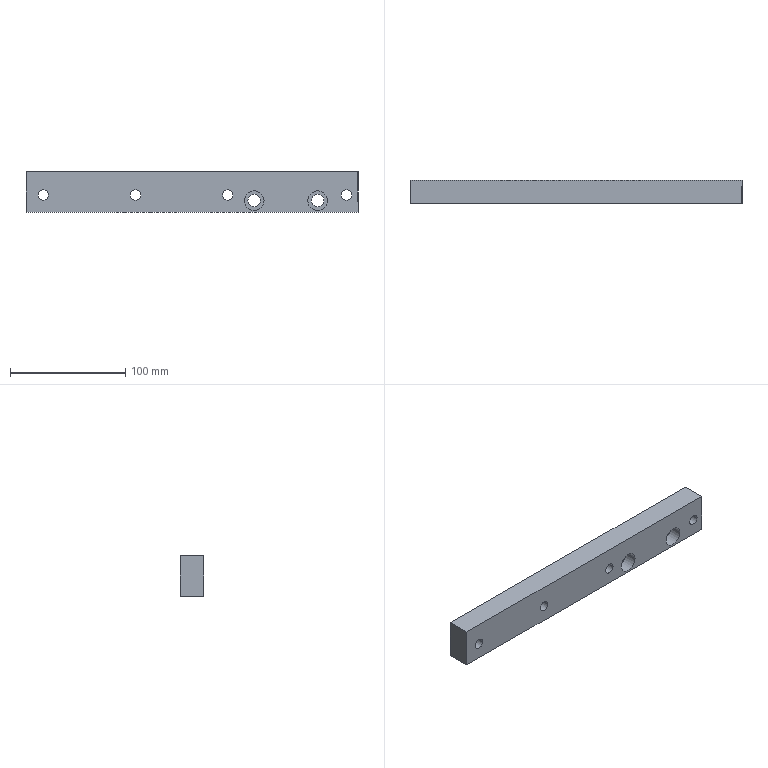Component | SolidWorks | SHYTJ-01-07-02ShimPlate-1 | 1 solid | 36 faces | box 288 x 20 x 35 mm | volume 185735 mm3 | cylinder 24 | plane 12 | commonest cylinder face diameters 15 x8 9 x8 11 x4 17 x4
STEP:
#1=COLOUR_RGB('',0.7922,0.8196,0.9333);
#2=FILL_AREA_STYLE_COLOUR('',#1);
#3=FILL_AREA_STYLE('',(#2));
#4=SURFACE_STYLE_FILL_AREA(#3);
#5=SURFACE_SIDE_STYLE('',(#4));
#6=SURFACE_STYLE_USAGE(.BOTH.,#5);
#7=PRESENTATION_STYLE_ASSIGNMENT((#6));
#8=CARTESIAN_POINT('',(-1.402,-6.471,9.311));
#9=VERTEX_POINT('',#8);
#10=CARTESIAN_POINT('',(-1.993,-6.471,9.311));
#11=VERTEX_POINT('',#10);
#12=CARTESIAN_POINT('',(-1.697,-6.471,9.311));
#13=DIRECTION('',(-0.,1.,0.));
#14=DIRECTION('',(-1.,0.,0.));
#15=AXIS2_PLACEMENT_3D('',#12,#13,#14);
#16=CIRCLE('',#15,0.2953);
#17=EDGE_CURVE('',#9,#11,#16,.T.);
#18=ORIENTED_EDGE('',*,*,#17,.F.);
#19=CARTESIAN_POINT('',(-1.402,-6.117,9.311));
#20=VERTEX_POINT('',#19);
#21=CARTESIAN_POINT('',(-1.402,-6.117,9.311));
#22=DIRECTION('',(-0.,1.,0.));
#23=VECTOR('',#22,39.37);
#24=LINE('',#21,#23);
#25=EDGE_CURVE('',#9,#20,#24,.T.);
#26=ORIENTED_EDGE('',*,*,#25,.T.);
#27=CARTESIAN_POINT('',(-1.993,-6.117,9.311));
#28=VERTEX_POINT('',#27);
#29=CARTESIAN_POINT('',(-1.697,-6.117,9.311));
#30=DIRECTION('',(-0.,1.,0.));
#31=DIRECTION('',(-1.,0.,0.));
#32=AXIS2_PLACEMENT_3D('',#29,#30,#31);
#33=CIRCLE('',#32,0.2953);
#34=EDGE_CURVE('',#20,#28,#33,.T.);
#35=ORIENTED_EDGE('',*,*,#34,.T.);
#36=CARTESIAN_POINT('',(-1.993,-6.117,9.311));
#37=DIRECTION('',(-0.,1.,0.));
#38=VECTOR('',#37,39.37);
#39=LINE('',#36,#38);
#40=EDGE_CURVE('',#11,#28,#39,.T.);
#41=ORIENTED_EDGE('',*,*,#40,.F.);
#42=EDGE_LOOP('',(#18,#26,#35,#41));
#43=FACE_OUTER_BOUND('',#42,.T.);
#44=CARTESIAN_POINT('',(-1.697,-6.117,9.311));
#45=DIRECTION('',(-0.,1.,0.));
#46=DIRECTION('',(-1.,0.,0.));
#47=AXIS2_PLACEMENT_3D('',#44,#45,#46);
#48=CYLINDRICAL_SURFACE('',#47,0.2953);
#49=ADVANCED_FACE('',(#43),#48,.F.);
#50=CARTESIAN_POINT('',(-1.52,-6.904,9.311));
#51=VERTEX_POINT('',#50);
#52=CARTESIAN_POINT('',(-1.875,-6.904,9.311));
#53=VERTEX_POINT('',#52);
#54=CARTESIAN_POINT('',(-1.697,-6.904,9.311));
#55=DIRECTION('',(-0.,1.,0.));
#56=DIRECTION('',(-1.,0.,0.));
#57=AXIS2_PLACEMENT_3D('',#54,#55,#56);
#58=CIRCLE('',#57,0.1772);
#59=EDGE_CURVE('',#51,#53,#58,.T.);
#60=ORIENTED_EDGE('',*,*,#59,.F.);
#61=CARTESIAN_POINT('',(-1.52,-6.471,9.311));
#62=VERTEX_POINT('',#61);
#63=CARTESIAN_POINT('',(-1.52,-6.117,9.311));
#64=DIRECTION('',(-0.,1.,0.));
#65=VECTOR('',#64,39.37);
#66=LINE('',#63,#65);
#67=EDGE_CURVE('',#51,#62,#66,.T.);
#68=ORIENTED_EDGE('',*,*,#67,.T.);
#69=CARTESIAN_POINT('',(-1.875,-6.471,9.311));
#70=VERTEX_POINT('',#69);
#71=CARTESIAN_POINT('',(-1.697,-6.471,9.311));
#72=DIRECTION('',(-0.,1.,0.));
#73=DIRECTION('',(-1.,0.,0.));
#74=AXIS2_PLACEMENT_3D('',#71,#72,#73);
#75=CIRCLE('',#74,0.1772);
#76=EDGE_CURVE('',#62,#70,#75,.T.);
#77=ORIENTED_EDGE('',*,*,#76,.T.);
#78=CARTESIAN_POINT('',(-1.875,-6.117,9.311));
#79=DIRECTION('',(-0.,1.,0.));
#80=VECTOR('',#79,39.37);
#81=LINE('',#78,#80);
#82=EDGE_CURVE('',#53,#70,#81,.T.);
#83=ORIENTED_EDGE('',*,*,#82,.F.);
#84=EDGE_LOOP('',(#60,#68,#77,#83));
#85=FACE_OUTER_BOUND('',#84,.T.);
#86=CARTESIAN_POINT('',(-1.697,-6.117,9.311));
#87=DIRECTION('',(-0.,1.,0.));
#88=DIRECTION('',(-1.,0.,0.));
#89=AXIS2_PLACEMENT_3D('',#86,#87,#88);
#90=CYLINDRICAL_SURFACE('',#89,0.1772);
#91=ADVANCED_FACE('',(#85),#90,.F.);
#92=CARTESIAN_POINT('',(1.747,-6.471,9.311));
#93=VERTEX_POINT('',#92);
#94=CARTESIAN_POINT('',(1.157,-6.471,9.311));
#95=VERTEX_POINT('',#94);
#96=CARTESIAN_POINT('',(1.452,-6.471,9.311));
#97=DIRECTION('',(-0.,1.,0.));
#98=DIRECTION('',(-1.,0.,0.));
#99=AXIS2_PLACEMENT_3D('',#96,#97,#98);
#100=CIRCLE('',#99,0.2953);
#101=EDGE_CURVE('',#93,#95,#100,.T.);
#102=ORIENTED_EDGE('',*,*,#101,.F.);
#103=CARTESIAN_POINT('',(1.747,-6.117,9.311));
#104=VERTEX_POINT('',#103);
#105=CARTESIAN_POINT('',(1.747,-6.117,9.311));
#106=DIRECTION('',(-0.,1.,0.));
#107=VECTOR('',#106,39.37);
#108=LINE('',#105,#107);
#109=EDGE_CURVE('',#93,#104,#108,.T.);
#110=ORIENTED_EDGE('',*,*,#109,.T.);
#111=CARTESIAN_POINT('',(1.157,-6.117,9.311));
#112=VERTEX_POINT('',#111);
#113=CARTESIAN_POINT('',(1.452,-6.117,9.311));
#114=DIRECTION('',(-0.,1.,0.));
#115=DIRECTION('',(-1.,0.,0.));
#116=AXIS2_PLACEMENT_3D('',#113,#114,#115);
#117=CIRCLE('',#116,0.2953);
#118=EDGE_CURVE('',#104,#112,#117,.T.);
#119=ORIENTED_EDGE('',*,*,#118,.T.);
#120=CARTESIAN_POINT('',(1.157,-6.117,9.311));
#121=DIRECTION('',(-0.,1.,0.));
#122=VECTOR('',#121,39.37);
#123=LINE('',#120,#122);
#124=EDGE_CURVE('',#95,#112,#123,.T.);
#125=ORIENTED_EDGE('',*,*,#124,.F.);
#126=EDGE_LOOP('',(#102,#110,#119,#125));
#127=FACE_OUTER_BOUND('',#126,.T.);
#128=CARTESIAN_POINT('',(1.452,-6.117,9.311));
#129=DIRECTION('',(-0.,1.,0.));
#130=DIRECTION('',(-1.,0.,0.));
#131=AXIS2_PLACEMENT_3D('',#128,#129,#130);
#132=CYLINDRICAL_SURFACE('',#131,0.2953);
#133=ADVANCED_FACE('',(#127),#132,.F.);
#134=CARTESIAN_POINT('',(1.629,-6.904,9.311));
#135=VERTEX_POINT('',#134);
#136=CARTESIAN_POINT('',(1.275,-6.904,9.311));
#137=VERTEX_POINT('',#136);
#138=CARTESIAN_POINT('',(1.452,-6.904,9.311));
#139=DIRECTION('',(-0.,1.,0.));
#140=DIRECTION('',(-1.,0.,0.));
#141=AXIS2_PLACEMENT_3D('',#138,#139,#140);
#142=CIRCLE('',#141,0.1772);
#143=EDGE_CURVE('',#135,#137,#142,.T.);
#144=ORIENTED_EDGE('',*,*,#143,.F.);
#145=CARTESIAN_POINT('',(1.629,-6.471,9.311));
#146=VERTEX_POINT('',#145);
#147=CARTESIAN_POINT('',(1.629,-6.117,9.311));
#148=DIRECTION('',(-0.,1.,0.));
#149=VECTOR('',#148,39.37);
#150=LINE('',#147,#149);
#151=EDGE_CURVE('',#135,#146,#150,.T.);
#152=ORIENTED_EDGE('',*,*,#151,.T.);
#153=CARTESIAN_POINT('',(1.275,-6.471,9.311));
#154=VERTEX_POINT('',#153);
#155=CARTESIAN_POINT('',(1.452,-6.471,9.311));
#156=DIRECTION('',(-0.,1.,0.));
#157=DIRECTION('',(-1.,0.,0.));
#158=AXIS2_PLACEMENT_3D('',#155,#156,#157);
#159=CIRCLE('',#158,0.1772);
#160=EDGE_CURVE('',#146,#154,#159,.T.);
#161=ORIENTED_EDGE('',*,*,#160,.T.);
#162=CARTESIAN_POINT('',(1.275,-6.117,9.311));
#163=DIRECTION('',(-0.,1.,0.));
#164=VECTOR('',#163,39.37);
#165=LINE('',#162,#164);
#166=EDGE_CURVE('',#137,#154,#165,.T.);
#167=ORIENTED_EDGE('',*,*,#166,.F.);
#168=EDGE_LOOP('',(#144,#152,#161,#167));
#169=FACE_OUTER_BOUND('',#168,.T.);
#170=CARTESIAN_POINT('',(1.452,-6.117,9.311));
#171=DIRECTION('',(-0.,1.,0.));
#172=DIRECTION('',(-1.,0.,0.));
#173=AXIS2_PLACEMENT_3D('',#170,#171,#172);
#174=CYLINDRICAL_SURFACE('',#173,0.1772);
#175=ADVANCED_FACE('',(#169),#174,.F.);
#176=CARTESIAN_POINT('',(4.897,-6.471,9.311));
#177=VERTEX_POINT('',#176);
#178=CARTESIAN_POINT('',(4.306,-6.471,9.311));
#179=VERTEX_POINT('',#178);
#180=CARTESIAN_POINT('',(4.602,-6.471,9.311));
#181=DIRECTION('',(-0.,1.,0.));
#182=DIRECTION('',(-1.,0.,0.));
#183=AXIS2_PLACEMENT_3D('',#180,#181,#182);
#184=CIRCLE('',#183,0.2953);
#185=EDGE_CURVE('',#177,#179,#184,.T.);
#186=ORIENTED_EDGE('',*,*,#185,.F.);
#187=CARTESIAN_POINT('',(4.897,-6.117,9.311));
#188=VERTEX_POINT('',#187);
#189=CARTESIAN_POINT('',(4.897,-6.117,9.311));
#190=DIRECTION('',(-0.,1.,0.));
#191=VECTOR('',#190,39.37);
#192=LINE('',#189,#191);
#193=EDGE_CURVE('',#177,#188,#192,.T.);
#194=ORIENTED_EDGE('',*,*,#193,.T.);
#195=CARTESIAN_POINT('',(4.306,-6.117,9.311));
#196=VERTEX_POINT('',#195);
#197=CARTESIAN_POINT('',(4.602,-6.117,9.311));
#198=DIRECTION('',(-0.,1.,0.));
#199=DIRECTION('',(-1.,0.,0.));
#200=AXIS2_PLACEMENT_3D('',#197,#198,#199);
#201=CIRCLE('',#200,0.2953);
#202=EDGE_CURVE('',#188,#196,#201,.T.);
#203=ORIENTED_EDGE('',*,*,#202,.T.);
#204=CARTESIAN_POINT('',(4.306,-6.117,9.311));
#205=DIRECTION('',(-0.,1.,0.));
#206=VECTOR('',#205,39.37);
#207=LINE('',#204,#206);
#208=EDGE_CURVE('',#179,#196,#207,.T.);
#209=ORIENTED_EDGE('',*,*,#208,.F.);
#210=EDGE_LOOP('',(#186,#194,#203,#209));
#211=FACE_OUTER_BOUND('',#210,.T.);
#212=CARTESIAN_POINT('',(4.602,-6.117,9.311));
#213=DIRECTION('',(-0.,1.,0.));
#214=DIRECTION('',(-1.,0.,0.));
#215=AXIS2_PLACEMENT_3D('',#212,#213,#214);
#216=CYLINDRICAL_SURFACE('',#215,0.2953);
#217=ADVANCED_FACE('',(#211),#216,.F.);
#218=CARTESIAN_POINT('',(4.779,-6.904,9.311));
#219=VERTEX_POINT('',#218);
#220=CARTESIAN_POINT('',(4.425,-6.904,9.311));
#221=VERTEX_POINT('',#220);
#222=CARTESIAN_POINT('',(4.602,-6.904,9.311));
#223=DIRECTION('',(-0.,1.,0.));
#224=DIRECTION('',(-1.,0.,0.));
#225=AXIS2_PLACEMENT_3D('',#222,#223,#224);
#226=CIRCLE('',#225,0.1772);
#227=EDGE_CURVE('',#219,#221,#226,.T.);
#228=ORIENTED_EDGE('',*,*,#227,.F.);
#229=CARTESIAN_POINT('',(4.779,-6.471,9.311));
#230=VERTEX_POINT('',#229);
#231=CARTESIAN_POINT('',(4.779,-6.117,9.311));
#232=DIRECTION('',(-0.,1.,0.));
#233=VECTOR('',#232,39.37);
#234=LINE('',#231,#233);
#235=EDGE_CURVE('',#219,#230,#234,.T.);
#236=ORIENTED_EDGE('',*,*,#235,.T.);
#237=CARTESIAN_POINT('',(4.425,-6.471,9.311));
#238=VERTEX_POINT('',#237);
#239=CARTESIAN_POINT('',(4.602,-6.471,9.311));
#240=DIRECTION('',(-0.,1.,0.));
#241=DIRECTION('',(-1.,0.,0.));
#242=AXIS2_PLACEMENT_3D('',#239,#240,#241);
#243=CIRCLE('',#242,0.1772);
#244=EDGE_CURVE('',#230,#238,#243,.T.);
#245=ORIENTED_EDGE('',*,*,#244,.T.);
#246=CARTESIAN_POINT('',(4.425,-6.117,9.311));
#247=DIRECTION('',(-0.,1.,0.));
#248=VECTOR('',#247,39.37);
#249=LINE('',#246,#248);
#250=EDGE_CURVE('',#221,#238,#249,.T.);
#251=ORIENTED_EDGE('',*,*,#250,.F.);
#252=EDGE_LOOP('',(#228,#236,#245,#251));
#253=FACE_OUTER_BOUND('',#252,.T.);
#254=CARTESIAN_POINT('',(4.602,-6.117,9.311));
#255=DIRECTION('',(-0.,1.,0.));
#256=DIRECTION('',(-1.,0.,0.));
#257=AXIS2_PLACEMENT_3D('',#254,#255,#256);
#258=CYLINDRICAL_SURFACE('',#257,0.1772);
#259=ADVANCED_FACE('',(#253),#258,.F.);
#260=CARTESIAN_POINT('',(8.952,-6.471,9.311));
#261=VERTEX_POINT('',#260);
#262=CARTESIAN_POINT('',(8.362,-6.471,9.311));
#263=VERTEX_POINT('',#262);
#264=CARTESIAN_POINT('',(8.657,-6.471,9.311));
#265=DIRECTION('',(-0.,1.,0.));
#266=DIRECTION('',(-1.,0.,0.));
#267=AXIS2_PLACEMENT_3D('',#264,#265,#266);
#268=CIRCLE('',#267,0.2953);
#269=EDGE_CURVE('',#261,#263,#268,.T.);
#270=ORIENTED_EDGE('',*,*,#269,.F.);
#271=CARTESIAN_POINT('',(8.952,-6.117,9.311));
#272=VERTEX_POINT('',#271);
#273=CARTESIAN_POINT('',(8.952,-6.117,9.311));
#274=DIRECTION('',(-0.,1.,0.));
#275=VECTOR('',#274,39.37);
#276=LINE('',#273,#275);
#277=EDGE_CURVE('',#261,#272,#276,.T.);
#278=ORIENTED_EDGE('',*,*,#277,.T.);
#279=CARTESIAN_POINT('',(8.362,-6.117,9.311));
#280=VERTEX_POINT('',#279);
#281=CARTESIAN_POINT('',(8.657,-6.117,9.311));
#282=DIRECTION('',(-0.,1.,0.));
#283=DIRECTION('',(-1.,0.,0.));
#284=AXIS2_PLACEMENT_3D('',#281,#282,#283);
#285=CIRCLE('',#284,0.2953);
#286=EDGE_CURVE('',#272,#280,#285,.T.);
#287=ORIENTED_EDGE('',*,*,#286,.T.);
#288=CARTESIAN_POINT('',(8.362,-6.117,9.311));
#289=DIRECTION('',(-0.,1.,0.));
#290=VECTOR('',#289,39.37);
#291=LINE('',#288,#290);
#292=EDGE_CURVE('',#263,#280,#291,.T.);
#293=ORIENTED_EDGE('',*,*,#292,.F.);
#294=EDGE_LOOP('',(#270,#278,#287,#293));
#295=FACE_OUTER_BOUND('',#294,.T.);
#296=CARTESIAN_POINT('',(8.657,-6.117,9.311));
#297=DIRECTION('',(-0.,1.,0.));
#298=DIRECTION('',(-1.,0.,0.));
#299=AXIS2_PLACEMENT_3D('',#296,#297,#298);
#300=CYLINDRICAL_SURFACE('',#299,0.2953);
#301=ADVANCED_FACE('',(#295),#300,.F.);
#302=CARTESIAN_POINT('',(8.834,-6.904,9.311));
#303=VERTEX_POINT('',#302);
#304=CARTESIAN_POINT('',(8.48,-6.904,9.311));
#305=VERTEX_POINT('',#304);
#306=CARTESIAN_POINT('',(8.657,-6.904,9.311));
#307=DIRECTION('',(-0.,1.,0.));
#308=DIRECTION('',(-1.,0.,0.));
#309=AXIS2_PLACEMENT_3D('',#306,#307,#308);
#310=CIRCLE('',#309,0.1772);
#311=EDGE_CURVE('',#303,#305,#310,.T.);
#312=ORIENTED_EDGE('',*,*,#311,.F.);
#313=CARTESIAN_POINT('',(8.834,-6.471,9.311));
#314=VERTEX_POINT('',#313);
#315=CARTESIAN_POINT('',(8.834,-6.117,9.311));
#316=DIRECTION('',(-0.,1.,0.));
#317=VECTOR('',#316,39.37);
#318=LINE('',#315,#317);
#319=EDGE_CURVE('',#303,#314,#318,.T.);
#320=ORIENTED_EDGE('',*,*,#319,.T.);
#321=CARTESIAN_POINT('',(8.48,-6.471,9.311));
#322=VERTEX_POINT('',#321);
#323=CARTESIAN_POINT('',(8.657,-6.471,9.311));
#324=DIRECTION('',(-0.,1.,0.));
#325=DIRECTION('',(-1.,0.,0.));
#326=AXIS2_PLACEMENT_3D('',#323,#324,#325);
#327=CIRCLE('',#326,0.1772);
#328=EDGE_CURVE('',#314,#322,#327,.T.);
#329=ORIENTED_EDGE('',*,*,#328,.T.);
#330=CARTESIAN_POINT('',(8.48,-6.117,9.311));
#331=DIRECTION('',(-0.,1.,0.));
#332=VECTOR('',#331,39.37);
#333=LINE('',#330,#332);
#334=EDGE_CURVE('',#305,#322,#333,.T.);
#335=ORIENTED_EDGE('',*,*,#334,.F.);
#336=EDGE_LOOP('',(#312,#320,#329,#335));
#337=FACE_OUTER_BOUND('',#336,.T.);
#338=CARTESIAN_POINT('',(8.657,-6.117,9.311));
#339=DIRECTION('',(-0.,1.,0.));
#340=DIRECTION('',(-1.,0.,0.));
#341=AXIS2_PLACEMENT_3D('',#338,#339,#340);
#342=CYLINDRICAL_SURFACE('',#341,0.1772);
#343=ADVANCED_FACE('',(#337),#342,.F.);
#344=CARTESIAN_POINT('',(7.456,-6.117,9.114));
#345=VERTEX_POINT('',#344);
#346=CARTESIAN_POINT('',(7.889,-6.117,9.114));
#347=VERTEX_POINT('',#346);
#348=CARTESIAN_POINT('',(7.673,-6.117,9.114));
#349=DIRECTION('',(0.,-1.,-0.));
#350=DIRECTION('',(1.,0.,0.));
#351=AXIS2_PLACEMENT_3D('',#348,#349,#350);
#352=CIRCLE('',#351,0.2165);
#353=EDGE_CURVE('',#345,#347,#352,.T.);
#354=ORIENTED_EDGE('',*,*,#353,.F.);
#355=CARTESIAN_POINT('',(7.456,-6.471,9.114));
#356=VERTEX_POINT('',#355);
#357=CARTESIAN_POINT('',(7.456,-6.904,9.114));
#358=DIRECTION('',(0.,-1.,-0.));
#359=VECTOR('',#358,39.37);
#360=LINE('',#357,#359);
#361=EDGE_CURVE('',#345,#356,#360,.T.);
#362=ORIENTED_EDGE('',*,*,#361,.T.);
#363=CARTESIAN_POINT('',(7.889,-6.471,9.114));
#364=VERTEX_POINT('',#363);
#365=CARTESIAN_POINT('',(7.673,-6.471,9.114));
#366=DIRECTION('',(0.,-1.,-0.));
#367=DIRECTION('',(1.,0.,0.));
#368=AXIS2_PLACEMENT_3D('',#365,#366,#367);
#369=CIRCLE('',#368,0.2165);
#370=EDGE_CURVE('',#356,#364,#369,.T.);
#371=ORIENTED_EDGE('',*,*,#370,.T.);
#372=CARTESIAN_POINT('',(7.889,-6.904,9.114));
#373=DIRECTION('',(0.,-1.,-0.));
#374=VECTOR('',#373,39.37);
#375=LINE('',#372,#374);
#376=EDGE_CURVE('',#347,#364,#375,.T.);
#377=ORIENTED_EDGE('',*,*,#376,.F.);
#378=EDGE_LOOP('',(#354,#362,#371,#377));
#379=FACE_OUTER_BOUND('',#378,.T.);
#380=CARTESIAN_POINT('',(7.673,-6.904,9.114));
#381=DIRECTION('',(0.,-1.,-0.));
#382=DIRECTION('',(1.,0.,0.));
#383=AXIS2_PLACEMENT_3D('',#380,#381,#382);
#384=CYLINDRICAL_SURFACE('',#383,0.2165);
#385=ADVANCED_FACE('',(#379),#384,.F.);
#386=CARTESIAN_POINT('',(5.291,-6.117,9.114));
#387=VERTEX_POINT('',#386);
#388=CARTESIAN_POINT('',(5.724,-6.117,9.114));
#389=VERTEX_POINT('',#388);
#390=CARTESIAN_POINT('',(5.507,-6.117,9.114));
#391=DIRECTION('',(0.,-1.,-0.));
#392=DIRECTION('',(1.,0.,0.));
#393=AXIS2_PLACEMENT_3D('',#390,#391,#392);
#394=CIRCLE('',#393,0.2165);
#395=EDGE_CURVE('',#387,#389,#394,.T.);
#396=ORIENTED_EDGE('',*,*,#395,.F.);
#397=CARTESIAN_POINT('',(5.291,-6.471,9.114));
#398=VERTEX_POINT('',#397);
#399=CARTESIAN_POINT('',(5.291,-6.904,9.114));
#400=DIRECTION('',(0.,-1.,-0.));
#401=VECTOR('',#400,39.37);
#402=LINE('',#399,#401);
#403=EDGE_CURVE('',#387,#398,#402,.T.);
#404=ORIENTED_EDGE('',*,*,#403,.T.);
#405=CARTESIAN_POINT('',(5.724,-6.471,9.114));
#406=VERTEX_POINT('',#405);
#407=CARTESIAN_POINT('',(5.507,-6.471,9.114));
#408=DIRECTION('',(0.,-1.,-0.));
#409=DIRECTION('',(1.,0.,0.));
#410=AXIS2_PLACEMENT_3D('',#407,#408,#409);
#411=CIRCLE('',#410,0.2165);
#412=EDGE_CURVE('',#398,#406,#411,.T.);
#413=ORIENTED_EDGE('',*,*,#412,.T.);
#414=CARTESIAN_POINT('',(5.724,-6.904,9.114));
#415=DIRECTION('',(0.,-1.,-0.));
#416=VECTOR('',#415,39.37);
#417=LINE('',#414,#416);
#418=EDGE_CURVE('',#389,#406,#417,.T.);
#419=ORIENTED_EDGE('',*,*,#418,.F.);
#420=EDGE_LOOP('',(#396,#404,#413,#419));
#421=FACE_OUTER_BOUND('',#420,.T.);
#422=CARTESIAN_POINT('',(5.507,-6.904,9.114));
#423=DIRECTION('',(0.,-1.,-0.));
#424=DIRECTION('',(1.,0.,0.));
#425=AXIS2_PLACEMENT_3D('',#422,#423,#424);
#426=CYLINDRICAL_SURFACE('',#425,0.2165);
#427=ADVANCED_FACE('',(#421),#426,.F.);
#428=CARTESIAN_POINT('',(7.338,-6.471,9.114));
#429=VERTEX_POINT('',#428);
#430=CARTESIAN_POINT('',(8.007,-6.471,9.114));
#431=VERTEX_POINT('',#430);
#432=CARTESIAN_POINT('',(7.673,-6.471,9.114));
#433=DIRECTION('',(0.,-1.,-0.));
#434=DIRECTION('',(1.,0.,0.));
#435=AXIS2_PLACEMENT_3D('',#432,#433,#434);
#436=CIRCLE('',#435,0.3346);
#437=EDGE_CURVE('',#429,#431,#436,.T.);
#438=ORIENTED_EDGE('',*,*,#437,.F.);
#439=CARTESIAN_POINT('',(7.338,-6.904,9.114));
#440=VERTEX_POINT('',#439);
#441=CARTESIAN_POINT('',(7.338,-6.904,9.114));
#442=DIRECTION('',(0.,-1.,-0.));
#443=VECTOR('',#442,39.37);
#444=LINE('',#441,#443);
#445=EDGE_CURVE('',#429,#440,#444,.T.);
#446=ORIENTED_EDGE('',*,*,#445,.T.);
#447=CARTESIAN_POINT('',(8.007,-6.904,9.114));
#448=VERTEX_POINT('',#447);
#449=CARTESIAN_POINT('',(7.673,-6.904,9.114));
#450=DIRECTION('',(0.,-1.,-0.));
#451=DIRECTION('',(1.,0.,0.));
#452=AXIS2_PLACEMENT_3D('',#449,#450,#451);
#453=CIRCLE('',#452,0.3346);
#454=EDGE_CURVE('',#440,#448,#453,.T.);
#455=ORIENTED_EDGE('',*,*,#454,.T.);
#456=CARTESIAN_POINT('',(8.007,-6.904,9.114));
#457=DIRECTION('',(0.,-1.,-0.));
#458=VECTOR('',#457,39.37);
#459=LINE('',#456,#458);
#460=EDGE_CURVE('',#431,#448,#459,.T.);
#461=ORIENTED_EDGE('',*,*,#460,.F.);
#462=EDGE_LOOP('',(#438,#446,#455,#461));
#463=FACE_OUTER_BOUND('',#462,.T.);
#464=CARTESIAN_POINT('',(7.673,-6.904,9.114));
#465=DIRECTION('',(0.,-1.,-0.));
#466=DIRECTION('',(1.,0.,0.));
#467=AXIS2_PLACEMENT_3D('',#464,#465,#466);
#468=CYLINDRICAL_SURFACE('',#467,0.3346);
#469=ADVANCED_FACE('',(#463),#468,.F.);
#470=CARTESIAN_POINT('',(5.173,-6.471,9.114));
#471=VERTEX_POINT('',#470);
#472=CARTESIAN_POINT('',(5.842,-6.471,9.114));
#473=VERTEX_POINT('',#472);
#474=CARTESIAN_POINT('',(5.507,-6.471,9.114));
#475=DIRECTION('',(0.,-1.,-0.));
#476=DIRECTION('',(1.,0.,0.));
#477=AXIS2_PLACEMENT_3D('',#474,#475,#476);
#478=CIRCLE('',#477,0.3346);
#479=EDGE_CURVE('',#471,#473,#478,.T.);
#480=ORIENTED_EDGE('',*,*,#479,.F.);
#481=CARTESIAN_POINT('',(5.173,-6.904,9.114));
#482=VERTEX_POINT('',#481);
#483=CARTESIAN_POINT('',(5.173,-6.904,9.114));
#484=DIRECTION('',(0.,-1.,-0.));
#485=VECTOR('',#484,39.37);
#486=LINE('',#483,#485);
#487=EDGE_CURVE('',#471,#482,#486,.T.);
#488=ORIENTED_EDGE('',*,*,#487,.T.);
#489=CARTESIAN_POINT('',(5.842,-6.904,9.114));
#490=VERTEX_POINT('',#489);
#491=CARTESIAN_POINT('',(5.507,-6.904,9.114));
#492=DIRECTION('',(0.,-1.,-0.));
#493=DIRECTION('',(1.,0.,0.));
#494=AXIS2_PLACEMENT_3D('',#491,#492,#493);
#495=CIRCLE('',#494,0.3346);
#496=EDGE_CURVE('',#482,#490,#495,.T.);
#497=ORIENTED_EDGE('',*,*,#496,.T.);
#498=CARTESIAN_POINT('',(5.842,-6.904,9.114));
#499=DIRECTION('',(0.,-1.,-0.));
#500=VECTOR('',#499,39.37);
#501=LINE('',#498,#500);
#502=EDGE_CURVE('',#473,#490,#501,.T.);
#503=ORIENTED_EDGE('',*,*,#502,.F.);
#504=EDGE_LOOP('',(#480,#488,#497,#503));
#505=FACE_OUTER_BOUND('',#504,.T.);
#506=CARTESIAN_POINT('',(5.507,-6.904,9.114));
#507=DIRECTION('',(0.,-1.,-0.));
#508=DIRECTION('',(1.,0.,0.));
#509=AXIS2_PLACEMENT_3D('',#506,#507,#508);
#510=CYLINDRICAL_SURFACE('',#509,0.3346);
#511=ADVANCED_FACE('',(#505),#510,.F.);
#512=CARTESIAN_POINT('',(5.507,-6.471,9.114));
#513=DIRECTION('',(0.,-1.,-0.));
#514=DIRECTION('',(1.,0.,0.));
#515=AXIS2_PLACEMENT_3D('',#512,#513,#514);
#516=CIRCLE('',#515,0.2165);
#517=EDGE_CURVE('',#406,#398,#516,.T.);
#518=ORIENTED_EDGE('',*,*,#517,.F.);
#519=ORIENTED_EDGE('',*,*,#412,.F.);
#520=EDGE_LOOP('',(#518,#519));
#521=FACE_BOUND('',#520,.T.);
#522=CARTESIAN_POINT('',(5.507,-6.471,9.114));
#523=DIRECTION('',(0.,-1.,-0.));
#524=DIRECTION('',(1.,0.,0.));
#525=AXIS2_PLACEMENT_3D('',#522,#523,#524);
#526=CIRCLE('',#525,0.3346);
#527=EDGE_CURVE('',#473,#471,#526,.T.);
#528=ORIENTED_EDGE('',*,*,#527,.T.);
#529=ORIENTED_EDGE('',*,*,#479,.T.);
#530=EDGE_LOOP('',(#528,#529));
#531=FACE_OUTER_BOUND('',#530,.T.);
#532=CARTESIAN_POINT('',(5.724,-6.471,9.114));
#533=DIRECTION('',(-0.,1.,0.));
#534=DIRECTION('',(-1.,-0.,-0.));
#535=AXIS2_PLACEMENT_3D('',#532,#533,#534);
#536=PLANE('',#535);
#537=ADVANCED_FACE('',(#521,#531),#536,.F.);
#538=CARTESIAN_POINT('',(7.673,-6.471,9.114));
#539=DIRECTION('',(0.,-1.,-0.));
#540=DIRECTION('',(1.,0.,0.));
#541=AXIS2_PLACEMENT_3D('',#538,#539,#540);
#542=CIRCLE('',#541,0.2165);
#543=EDGE_CURVE('',#364,#356,#542,.T.);
#544=ORIENTED_EDGE('',*,*,#543,.F.);
#545=ORIENTED_EDGE('',*,*,#370,.F.);
#546=EDGE_LOOP('',(#544,#545));
#547=FACE_BOUND('',#546,.T.);
#548=CARTESIAN_POINT('',(7.673,-6.471,9.114));
#549=DIRECTION('',(0.,-1.,-0.));
#550=DIRECTION('',(1.,0.,0.));
#551=AXIS2_PLACEMENT_3D('',#548,#549,#550);
#552=CIRCLE('',#551,0.3346);
#553=EDGE_CURVE('',#431,#429,#552,.T.);
#554=ORIENTED_EDGE('',*,*,#553,.T.);
#555=ORIENTED_EDGE('',*,*,#437,.T.);
#556=EDGE_LOOP('',(#554,#555));
#557=FACE_OUTER_BOUND('',#556,.T.);
#558=CARTESIAN_POINT('',(7.889,-6.471,9.114));
#559=DIRECTION('',(-0.,1.,0.));
#560=DIRECTION('',(-1.,-0.,-0.));
#561=AXIS2_PLACEMENT_3D('',#558,#559,#560);
#562=PLANE('',#561);
#563=ADVANCED_FACE('',(#547,#557),#562,.F.);
#564=ORIENTED_EDGE('',*,*,#487,.F.);
#565=ORIENTED_EDGE('',*,*,#527,.F.);
#566=ORIENTED_EDGE('',*,*,#502,.T.);
#567=CARTESIAN_POINT('',(5.507,-6.904,9.114));
#568=DIRECTION('',(0.,-1.,-0.));
#569=DIRECTION('',(1.,0.,0.));
#570=AXIS2_PLACEMENT_3D('',#567,#568,#569);
#571=CIRCLE('',#570,0.3346);
#572=EDGE_CURVE('',#490,#482,#571,.T.);
#573=ORIENTED_EDGE('',*,*,#572,.T.);
#574=EDGE_LOOP('',(#564,#565,#566,#573));
#575=FACE_OUTER_BOUND('',#574,.T.);
#576=CARTESIAN_POINT('',(5.507,-6.904,9.114));
#577=DIRECTION('',(0.,-1.,-0.));
#578=DIRECTION('',(1.,0.,0.));
#579=AXIS2_PLACEMENT_3D('',#576,#577,#578);
#580=CYLINDRICAL_SURFACE('',#579,0.3346);
#581=ADVANCED_FACE('',(#575),#580,.F.);
#582=ORIENTED_EDGE('',*,*,#445,.F.);
#583=ORIENTED_EDGE('',*,*,#553,.F.);
#584=ORIENTED_EDGE('',*,*,#460,.T.);
#585=CARTESIAN_POINT('',(7.673,-6.904,9.114));
#586=DIRECTION('',(0.,-1.,-0.));
#587=DIRECTION('',(1.,0.,0.));
#588=AXIS2_PLACEMENT_3D('',#585,#586,#587);
#589=CIRCLE('',#588,0.3346);
#590=EDGE_CURVE('',#448,#440,#589,.T.);
#591=ORIENTED_EDGE('',*,*,#590,.T.);
#592=EDGE_LOOP('',(#582,#583,#584,#591));
#593=FACE_OUTER_BOUND('',#592,.T.);
#594=CARTESIAN_POINT('',(7.673,-6.904,9.114));
#595=DIRECTION('',(0.,-1.,-0.));
#596=DIRECTION('',(1.,0.,0.));
#597=AXIS2_PLACEMENT_3D('',#594,#595,#596);
#598=CYLINDRICAL_SURFACE('',#597,0.3346);
#599=ADVANCED_FACE('',(#593),#598,.F.);
#600=ORIENTED_EDGE('',*,*,#403,.F.);
#601=CARTESIAN_POINT('',(5.507,-6.117,9.114));
#602=DIRECTION('',(0.,-1.,-0.));
#603=DIRECTION('',(1.,0.,0.));
#604=AXIS2_PLACEMENT_3D('',#601,#602,#603);
#605=CIRCLE('',#604,0.2165);
#606=EDGE_CURVE('',#389,#387,#605,.T.);
#607=ORIENTED_EDGE('',*,*,#606,.F.);
#608=ORIENTED_EDGE('',*,*,#418,.T.);
#609=ORIENTED_EDGE('',*,*,#517,.T.);
#610=EDGE_LOOP('',(#600,#607,#608,#609));
#611=FACE_OUTER_BOUND('',#610,.T.);
#612=CARTESIAN_POINT('',(5.507,-6.904,9.114));
#613=DIRECTION('',(0.,-1.,-0.));
#614=DIRECTION('',(1.,0.,0.));
#615=AXIS2_PLACEMENT_3D('',#612,#613,#614);
#616=CYLINDRICAL_SURFACE('',#615,0.2165);
#617=ADVANCED_FACE('',(#611),#616,.F.);
#618=ORIENTED_EDGE('',*,*,#361,.F.);
#619=CARTESIAN_POINT('',(7.673,-6.117,9.114));
#620=DIRECTION('',(0.,-1.,-0.));
#621=DIRECTION('',(1.,0.,0.));
#622=AXIS2_PLACEMENT_3D('',#619,#620,#621);
#623=CIRCLE('',#622,0.2165);
#624=EDGE_CURVE('',#347,#345,#623,.T.);
#625=ORIENTED_EDGE('',*,*,#624,.F.);
#626=ORIENTED_EDGE('',*,*,#376,.T.);
#627=ORIENTED_EDGE('',*,*,#543,.T.);
#628=EDGE_LOOP('',(#618,#625,#626,#627));
#629=FACE_OUTER_BOUND('',#628,.T.);
#630=CARTESIAN_POINT('',(7.673,-6.904,9.114));
#631=DIRECTION('',(0.,-1.,-0.));
#632=DIRECTION('',(1.,0.,0.));
#633=AXIS2_PLACEMENT_3D('',#630,#631,#632);
#634=CYLINDRICAL_SURFACE('',#633,0.2165);
#635=ADVANCED_FACE('',(#629),#634,.F.);
#636=CARTESIAN_POINT('',(-2.288,-6.117,8.72));
#637=VERTEX_POINT('',#636);
#638=CARTESIAN_POINT('',(9.051,-6.117,8.72));
#639=VERTEX_POINT('',#638);
#640=CARTESIAN_POINT('',(-2.288,-6.117,8.72));
#641=DIRECTION('',(1.,0.,0.));
#642=VECTOR('',#641,39.37);
#643=LINE('',#640,#642);
#644=EDGE_CURVE('',#637,#639,#643,.T.);
#645=ORIENTED_EDGE('',*,*,#644,.T.);
#646=CARTESIAN_POINT('',(9.051,-6.904,8.72));
#647=VERTEX_POINT('',#646);
#648=CARTESIAN_POINT('',(9.051,-6.904,8.72));
#649=DIRECTION('',(-0.,1.,0.));
#650=VECTOR('',#649,39.37);
#651=LINE('',#648,#650);
#652=EDGE_CURVE('',#647,#639,#651,.T.);
#653=ORIENTED_EDGE('',*,*,#652,.F.);
#654=CARTESIAN_POINT('',(-2.288,-6.904,8.72));
#655=VERTEX_POINT('',#654);
#656=CARTESIAN_POINT('',(-2.288,-6.904,8.72));
#657=DIRECTION('',(1.,0.,0.));
#658=VECTOR('',#657,39.37);
#659=LINE('',#656,#658);
#660=EDGE_CURVE('',#655,#647,#659,.T.);
#661=ORIENTED_EDGE('',*,*,#660,.F.);
#662=CARTESIAN_POINT('',(-2.288,-6.904,8.72));
#663=DIRECTION('',(-0.,1.,0.));
#664=VECTOR('',#663,39.37);
#665=LINE('',#662,#664);
#666=EDGE_CURVE('',#655,#637,#665,.T.);
#667=ORIENTED_EDGE('',*,*,#666,.T.);
#668=EDGE_LOOP('',(#645,#653,#661,#667));
#669=FACE_OUTER_BOUND('',#668,.T.);
#670=CARTESIAN_POINT('',(-2.288,-6.904,8.72));
#671=DIRECTION('',(-0.,-0.,1.));
#672=DIRECTION('',(0.,-1.,-0.));
#673=AXIS2_PLACEMENT_3D('',#670,#671,#672);
#674=PLANE('',#673);
#675=ADVANCED_FACE('',(#669),#674,.F.);
#676=CARTESIAN_POINT('',(-1.697,-6.904,9.311));
#677=DIRECTION('',(-0.,1.,0.));
#678=DIRECTION('',(-1.,0.,0.));
#679=AXIS2_PLACEMENT_3D('',#676,#677,#678);
#680=CIRCLE('',#679,0.1772);
#681=EDGE_CURVE('',#53,#51,#680,.T.);
#682=ORIENTED_EDGE('',*,*,#681,.T.);
#683=ORIENTED_EDGE('',*,*,#59,.T.);
#684=EDGE_LOOP('',(#682,#683));
#685=FACE_BOUND('',#684,.T.);
#686=CARTESIAN_POINT('',(1.452,-6.904,9.311));
#687=DIRECTION('',(-0.,1.,0.));
#688=DIRECTION('',(-1.,0.,0.));
#689=AXIS2_PLACEMENT_3D('',#686,#687,#688);
#690=CIRCLE('',#689,0.1772);
#691=EDGE_CURVE('',#137,#135,#690,.T.);
#692=ORIENTED_EDGE('',*,*,#691,.T.);
#693=ORIENTED_EDGE('',*,*,#143,.T.);
#694=EDGE_LOOP('',(#692,#693));
#695=FACE_BOUND('',#694,.T.);
#696=CARTESIAN_POINT('',(4.602,-6.904,9.311));
#697=DIRECTION('',(-0.,1.,0.));
#698=DIRECTION('',(-1.,0.,0.));
#699=AXIS2_PLACEMENT_3D('',#696,#697,#698);
#700=CIRCLE('',#699,0.1772);
#701=EDGE_CURVE('',#221,#219,#700,.T.);
#702=ORIENTED_EDGE('',*,*,#701,.T.);
#703=ORIENTED_EDGE('',*,*,#227,.T.);
#704=EDGE_LOOP('',(#702,#703));
#705=FACE_BOUND('',#704,.T.);
#706=CARTESIAN_POINT('',(8.657,-6.904,9.311));
#707=DIRECTION('',(-0.,1.,0.));
#708=DIRECTION('',(-1.,0.,0.));
#709=AXIS2_PLACEMENT_3D('',#706,#707,#708);
#710=CIRCLE('',#709,0.1772);
#711=EDGE_CURVE('',#305,#303,#710,.T.);
#712=ORIENTED_EDGE('',*,*,#711,.T.);
#713=ORIENTED_EDGE('',*,*,#311,.T.);
#714=EDGE_LOOP('',(#712,#713));
#715=FACE_BOUND('',#714,.T.);
#716=ORIENTED_EDGE('',*,*,#590,.F.);
#717=ORIENTED_EDGE('',*,*,#454,.F.);
#718=EDGE_LOOP('',(#716,#717));
#719=FACE_BOUND('',#718,.T.);
#720=ORIENTED_EDGE('',*,*,#572,.F.);
#721=ORIENTED_EDGE('',*,*,#496,.F.);
#722=EDGE_LOOP('',(#720,#721));
#723=FACE_BOUND('',#722,.T.);
#724=CARTESIAN_POINT('',(9.051,-6.904,10.098));
#725=VERTEX_POINT('',#724);
#726=CARTESIAN_POINT('',(9.051,-6.904,8.72));
#727=DIRECTION('',(-0.,-0.,1.));
#728=VECTOR('',#727,39.37);
#729=LINE('',#726,#728);
#730=EDGE_CURVE('',#647,#725,#729,.T.);
#731=ORIENTED_EDGE('',*,*,#730,.T.);
#732=CARTESIAN_POINT('',(-2.288,-6.904,10.098));
#733=VERTEX_POINT('',#732);
#734=CARTESIAN_POINT('',(-2.585,-6.904,10.098));
#735=DIRECTION('',(1.,0.,0.));
#736=VECTOR('',#735,39.37);
#737=LINE('',#734,#736);
#738=EDGE_CURVE('',#733,#725,#737,.T.);
#739=ORIENTED_EDGE('',*,*,#738,.F.);
#740=CARTESIAN_POINT('',(-2.288,-6.904,8.72));
#741=DIRECTION('',(0.,0.,-1.));
#742=VECTOR('',#741,39.37);
#743=LINE('',#740,#742);
#744=EDGE_CURVE('',#733,#655,#743,.T.);
#745=ORIENTED_EDGE('',*,*,#744,.T.);
#746=ORIENTED_EDGE('',*,*,#660,.T.);
#747=EDGE_LOOP('',(#731,#739,#745,#746));
#748=FACE_OUTER_BOUND('',#747,.T.);
#749=CARTESIAN_POINT('',(-2.288,-6.904,8.72));
#750=DIRECTION('',(-0.,1.,0.));
#751=DIRECTION('',(-1.,-0.,-0.));
#752=AXIS2_PLACEMENT_3D('',#749,#750,#751);
#753=PLANE('',#752);
#754=ADVANCED_FACE('',(#685,#695,#705,#715,#719,#723,#748),#753,.F.);
#755=CARTESIAN_POINT('',(-1.697,-6.117,9.311));
#756=DIRECTION('',(-0.,1.,0.));
#757=DIRECTION('',(-1.,0.,0.));
#758=AXIS2_PLACEMENT_3D('',#755,#756,#757);
#759=CIRCLE('',#758,0.2953);
#760=EDGE_CURVE('',#28,#20,#759,.T.);
#761=ORIENTED_EDGE('',*,*,#760,.F.);
#762=ORIENTED_EDGE('',*,*,#34,.F.);
#763=EDGE_LOOP('',(#761,#762));
#764=FACE_BOUND('',#763,.T.);
#765=CARTESIAN_POINT('',(1.452,-6.117,9.311));
#766=DIRECTION('',(-0.,1.,0.));
#767=DIRECTION('',(-1.,0.,0.));
#768=AXIS2_PLACEMENT_3D('',#765,#766,#767);
#769=CIRCLE('',#768,0.2953);
#770=EDGE_CURVE('',#112,#104,#769,.T.);
#771=ORIENTED_EDGE('',*,*,#770,.F.);
#772=ORIENTED_EDGE('',*,*,#118,.F.);
#773=EDGE_LOOP('',(#771,#772));
#774=FACE_BOUND('',#773,.T.);
#775=CARTESIAN_POINT('',(4.602,-6.117,9.311));
#776=DIRECTION('',(-0.,1.,0.));
#777=DIRECTION('',(-1.,0.,0.));
#778=AXIS2_PLACEMENT_3D('',#775,#776,#777);
#779=CIRCLE('',#778,0.2953);
#780=EDGE_CURVE('',#196,#188,#779,.T.);
#781=ORIENTED_EDGE('',*,*,#780,.F.);
#782=ORIENTED_EDGE('',*,*,#202,.F.);
#783=EDGE_LOOP('',(#781,#782));
#784=FACE_BOUND('',#783,.T.);
#785=CARTESIAN_POINT('',(8.657,-6.117,9.311));
#786=DIRECTION('',(-0.,1.,0.));
#787=DIRECTION('',(-1.,0.,0.));
#788=AXIS2_PLACEMENT_3D('',#785,#786,#787);
#789=CIRCLE('',#788,0.2953);
#790=EDGE_CURVE('',#280,#272,#789,.T.);
#791=ORIENTED_EDGE('',*,*,#790,.F.);
#792=ORIENTED_EDGE('',*,*,#286,.F.);
#793=EDGE_LOOP('',(#791,#792));
#794=FACE_BOUND('',#793,.T.);
#795=CARTESIAN_POINT('',(9.051,-6.117,10.098));
#796=VERTEX_POINT('',#795);
#797=CARTESIAN_POINT('',(-2.288,-6.117,10.098));
#798=VERTEX_POINT('',#797);
#799=CARTESIAN_POINT('',(-2.288,-6.117,10.098));
#800=DIRECTION('',(-1.,-0.,-0.));
#801=VECTOR('',#800,39.37);
#802=LINE('',#799,#801);
#803=EDGE_CURVE('',#796,#798,#802,.T.);
#804=ORIENTED_EDGE('',*,*,#803,.F.);
#805=CARTESIAN_POINT('',(9.051,-6.117,8.72));
#806=DIRECTION('',(-0.,-0.,1.));
#807=VECTOR('',#806,39.37);
#808=LINE('',#805,#807);
#809=EDGE_CURVE('',#639,#796,#808,.T.);
#810=ORIENTED_EDGE('',*,*,#809,.F.);
#811=ORIENTED_EDGE('',*,*,#644,.F.);
#812=CARTESIAN_POINT('',(-2.288,-6.117,8.72));
#813=DIRECTION('',(0.,0.,-1.));
#814=VECTOR('',#813,39.37);
#815=LINE('',#812,#814);
#816=EDGE_CURVE('',#798,#637,#815,.T.);
#817=ORIENTED_EDGE('',*,*,#816,.F.);
#818=EDGE_LOOP('',(#804,#810,#811,#817));
#819=FACE_OUTER_BOUND('',#818,.T.);
#820=ORIENTED_EDGE('',*,*,#624,.T.);
#821=ORIENTED_EDGE('',*,*,#353,.T.);
#822=EDGE_LOOP('',(#820,#821));
#823=FACE_BOUND('',#822,.T.);
#824=ORIENTED_EDGE('',*,*,#606,.T.);
#825=ORIENTED_EDGE('',*,*,#395,.T.);
#826=EDGE_LOOP('',(#824,#825));
#827=FACE_BOUND('',#826,.T.);
#828=CARTESIAN_POINT('',(-2.288,-6.117,8.72));
#829=DIRECTION('',(-0.,1.,0.));
#830=DIRECTION('',(-1.,-0.,-0.));
#831=AXIS2_PLACEMENT_3D('',#828,#829,#830);
#832=PLANE('',#831);
#833=ADVANCED_FACE('',(#764,#774,#784,#794,#819,#823,#827),#832,.T.);
#834=ORIENTED_EDGE('',*,*,#809,.T.);
#835=CARTESIAN_POINT('',(9.051,-6.904,10.098));
#836=DIRECTION('',(0.,-1.,-0.));
#837=VECTOR('',#836,39.37);
#838=LINE('',#835,#837);
#839=EDGE_CURVE('',#796,#725,#838,.T.);
#840=ORIENTED_EDGE('',*,*,#839,.T.);
#841=ORIENTED_EDGE('',*,*,#730,.F.);
#842=ORIENTED_EDGE('',*,*,#652,.T.);
#843=EDGE_LOOP('',(#834,#840,#841,#842));
#844=FACE_OUTER_BOUND('',#843,.T.);
#845=CARTESIAN_POINT('',(9.051,-6.904,8.72));
#846=DIRECTION('',(-1.,-0.,-0.));
#847=DIRECTION('',(0.,-1.,-0.));
#848=AXIS2_PLACEMENT_3D('',#845,#846,#847);
#849=PLANE('',#848);
#850=ADVANCED_FACE('',(#844),#849,.F.);
#851=ORIENTED_EDGE('',*,*,#744,.F.);
#852=CARTESIAN_POINT('',(-2.288,-6.904,10.098));
#853=DIRECTION('',(-0.,1.,0.));
#854=VECTOR('',#853,39.37);
#855=LINE('',#852,#854);
#856=EDGE_CURVE('',#733,#798,#855,.T.);
#857=ORIENTED_EDGE('',*,*,#856,.T.);
#858=ORIENTED_EDGE('',*,*,#816,.T.);
#859=ORIENTED_EDGE('',*,*,#666,.F.);
#860=EDGE_LOOP('',(#851,#857,#858,#859));
#861=FACE_OUTER_BOUND('',#860,.T.);
#862=CARTESIAN_POINT('',(-2.288,-6.904,8.72));
#863=DIRECTION('',(1.,0.,0.));
#864=DIRECTION('',(-0.,1.,0.));
#865=AXIS2_PLACEMENT_3D('',#862,#863,#864);
#866=PLANE('',#865);
#867=ADVANCED_FACE('',(#861),#866,.F.);
#868=ORIENTED_EDGE('',*,*,#738,.T.);
#869=ORIENTED_EDGE('',*,*,#839,.F.);
#870=ORIENTED_EDGE('',*,*,#803,.T.);
#871=ORIENTED_EDGE('',*,*,#856,.F.);
#872=EDGE_LOOP('',(#868,#869,#870,#871));
#873=FACE_OUTER_BOUND('',#872,.T.);
#874=CARTESIAN_POINT('',(-2.585,-6.117,10.098));
#875=DIRECTION('',(0.,0.,-1.));
#876=DIRECTION('',(-0.,1.,0.));
#877=AXIS2_PLACEMENT_3D('',#874,#875,#876);
#878=PLANE('',#877);
#879=ADVANCED_FACE('',(#873),#878,.F.);
#880=ORIENTED_EDGE('',*,*,#319,.F.);
#881=ORIENTED_EDGE('',*,*,#711,.F.);
#882=ORIENTED_EDGE('',*,*,#334,.T.);
#883=CARTESIAN_POINT('',(8.657,-6.471,9.311));
#884=DIRECTION('',(-0.,1.,0.));
#885=DIRECTION('',(-1.,0.,0.));
#886=AXIS2_PLACEMENT_3D('',#883,#884,#885);
#887=CIRCLE('',#886,0.1772);
#888=EDGE_CURVE('',#322,#314,#887,.T.);
#889=ORIENTED_EDGE('',*,*,#888,.T.);
#890=EDGE_LOOP('',(#880,#881,#882,#889));
#891=FACE_OUTER_BOUND('',#890,.T.);
#892=CARTESIAN_POINT('',(8.657,-6.117,9.311));
#893=DIRECTION('',(-0.,1.,0.));
#894=DIRECTION('',(-1.,0.,0.));
#895=AXIS2_PLACEMENT_3D('',#892,#893,#894);
#896=CYLINDRICAL_SURFACE('',#895,0.1772);
#897=ADVANCED_FACE('',(#891),#896,.F.);
#898=ORIENTED_EDGE('',*,*,#888,.F.);
#899=ORIENTED_EDGE('',*,*,#328,.F.);
#900=EDGE_LOOP('',(#898,#899));
#901=FACE_BOUND('',#900,.T.);
#902=CARTESIAN_POINT('',(8.657,-6.471,9.311));
#903=DIRECTION('',(-0.,1.,0.));
#904=DIRECTION('',(-1.,0.,0.));
#905=AXIS2_PLACEMENT_3D('',#902,#903,#904);
#906=CIRCLE('',#905,0.2953);
#907=EDGE_CURVE('',#263,#261,#906,.T.);
#908=ORIENTED_EDGE('',*,*,#907,.T.);
#909=ORIENTED_EDGE('',*,*,#269,.T.);
#910=EDGE_LOOP('',(#908,#909));
#911=FACE_OUTER_BOUND('',#910,.T.);
#912=CARTESIAN_POINT('',(8.834,-6.471,9.311));
#913=DIRECTION('',(0.,-1.,-0.));
#914=DIRECTION('',(1.,0.,0.));
#915=AXIS2_PLACEMENT_3D('',#912,#913,#914);
#916=PLANE('',#915);
#917=ADVANCED_FACE('',(#901,#911),#916,.F.);
#918=ORIENTED_EDGE('',*,*,#277,.F.);
#919=ORIENTED_EDGE('',*,*,#907,.F.);
#920=ORIENTED_EDGE('',*,*,#292,.T.);
#921=ORIENTED_EDGE('',*,*,#790,.T.);
#922=EDGE_LOOP('',(#918,#919,#920,#921));
#923=FACE_OUTER_BOUND('',#922,.T.);
#924=CARTESIAN_POINT('',(8.657,-6.117,9.311));
#925=DIRECTION('',(-0.,1.,0.));
#926=DIRECTION('',(-1.,0.,0.));
#927=AXIS2_PLACEMENT_3D('',#924,#925,#926);
#928=CYLINDRICAL_SURFACE('',#927,0.2953);
#929=ADVANCED_FACE('',(#923),#928,.F.);
#930=ORIENTED_EDGE('',*,*,#235,.F.);
#931=ORIENTED_EDGE('',*,*,#701,.F.);
#932=ORIENTED_EDGE('',*,*,#250,.T.);
#933=CARTESIAN_POINT('',(4.602,-6.471,9.311));
#934=DIRECTION('',(-0.,1.,0.));
#935=DIRECTION('',(-1.,0.,0.));
#936=AXIS2_PLACEMENT_3D('',#933,#934,#935);
#937=CIRCLE('',#936,0.1772);
#938=EDGE_CURVE('',#238,#230,#937,.T.);
#939=ORIENTED_EDGE('',*,*,#938,.T.);
#940=EDGE_LOOP('',(#930,#931,#932,#939));
#941=FACE_OUTER_BOUND('',#940,.T.);
#942=CARTESIAN_POINT('',(4.602,-6.117,9.311));
#943=DIRECTION('',(-0.,1.,0.));
#944=DIRECTION('',(-1.,0.,0.));
#945=AXIS2_PLACEMENT_3D('',#942,#943,#944);
#946=CYLINDRICAL_SURFACE('',#945,0.1772);
#947=ADVANCED_FACE('',(#941),#946,.F.);
#948=ORIENTED_EDGE('',*,*,#938,.F.);
#949=ORIENTED_EDGE('',*,*,#244,.F.);
#950=EDGE_LOOP('',(#948,#949));
#951=FACE_BOUND('',#950,.T.);
#952=CARTESIAN_POINT('',(4.602,-6.471,9.311));
#953=DIRECTION('',(-0.,1.,0.));
#954=DIRECTION('',(-1.,0.,0.));
#955=AXIS2_PLACEMENT_3D('',#952,#953,#954);
#956=CIRCLE('',#955,0.2953);
#957=EDGE_CURVE('',#179,#177,#956,.T.);
#958=ORIENTED_EDGE('',*,*,#957,.T.);
#959=ORIENTED_EDGE('',*,*,#185,.T.);
#960=EDGE_LOOP('',(#958,#959));
#961=FACE_OUTER_BOUND('',#960,.T.);
#962=CARTESIAN_POINT('',(4.779,-6.471,9.311));
#963=DIRECTION('',(0.,-1.,-0.));
#964=DIRECTION('',(1.,0.,0.));
#965=AXIS2_PLACEMENT_3D('',#962,#963,#964);
#966=PLANE('',#965);
#967=ADVANCED_FACE('',(#951,#961),#966,.F.);
#968=ORIENTED_EDGE('',*,*,#193,.F.);
#969=ORIENTED_EDGE('',*,*,#957,.F.);
#970=ORIENTED_EDGE('',*,*,#208,.T.);
#971=ORIENTED_EDGE('',*,*,#780,.T.);
#972=EDGE_LOOP('',(#968,#969,#970,#971));
#973=FACE_OUTER_BOUND('',#972,.T.);
#974=CARTESIAN_POINT('',(4.602,-6.117,9.311));
#975=DIRECTION('',(-0.,1.,0.));
#976=DIRECTION('',(-1.,0.,0.));
#977=AXIS2_PLACEMENT_3D('',#974,#975,#976);
#978=CYLINDRICAL_SURFACE('',#977,0.2953);
#979=ADVANCED_FACE('',(#973),#978,.F.);
#980=ORIENTED_EDGE('',*,*,#151,.F.);
#981=ORIENTED_EDGE('',*,*,#691,.F.);
#982=ORIENTED_EDGE('',*,*,#166,.T.);
#983=CARTESIAN_POINT('',(1.452,-6.471,9.311));
#984=DIRECTION('',(-0.,1.,0.));
#985=DIRECTION('',(-1.,0.,0.));
#986=AXIS2_PLACEMENT_3D('',#983,#984,#985);
#987=CIRCLE('',#986,0.1772);
#988=EDGE_CURVE('',#154,#146,#987,.T.);
#989=ORIENTED_EDGE('',*,*,#988,.T.);
#990=EDGE_LOOP('',(#980,#981,#982,#989));
#991=FACE_OUTER_BOUND('',#990,.T.);
#992=CARTESIAN_POINT('',(1.452,-6.117,9.311));
#993=DIRECTION('',(-0.,1.,0.));
#994=DIRECTION('',(-1.,0.,0.));
#995=AXIS2_PLACEMENT_3D('',#992,#993,#994);
#996=CYLINDRICAL_SURFACE('',#995,0.1772);
#997=ADVANCED_FACE('',(#991),#996,.F.);
#998=ORIENTED_EDGE('',*,*,#988,.F.);
#999=ORIENTED_EDGE('',*,*,#160,.F.);
#1000=EDGE_LOOP('',(#998,#999));
#1001=FACE_BOUND('',#1000,.T.);
#1002=CARTESIAN_POINT('',(1.452,-6.471,9.311));
#1003=DIRECTION('',(-0.,1.,0.));
#1004=DIRECTION('',(-1.,0.,0.));
#1005=AXIS2_PLACEMENT_3D('',#1002,#1003,#1004);
#1006=CIRCLE('',#1005,0.2953);
#1007=EDGE_CURVE('',#95,#93,#1006,.T.);
#1008=ORIENTED_EDGE('',*,*,#1007,.T.);
#1009=ORIENTED_EDGE('',*,*,#101,.T.);
#1010=EDGE_LOOP('',(#1008,#1009));
#1011=FACE_OUTER_BOUND('',#1010,.T.);
#1012=CARTESIAN_POINT('',(1.629,-6.471,9.311));
#1013=DIRECTION('',(0.,-1.,-0.));
#1014=DIRECTION('',(1.,0.,0.));
#1015=AXIS2_PLACEMENT_3D('',#1012,#1013,#1014);
#1016=PLANE('',#1015);
#1017=ADVANCED_FACE('',(#1001,#1011),#1016,.F.);
#1018=ORIENTED_EDGE('',*,*,#109,.F.);
#1019=ORIENTED_EDGE('',*,*,#1007,.F.);
#1020=ORIENTED_EDGE('',*,*,#124,.T.);
#1021=ORIENTED_EDGE('',*,*,#770,.T.);
#1022=EDGE_LOOP('',(#1018,#1019,#1020,#1021));
#1023=FACE_OUTER_BOUND('',#1022,.T.);
#1024=CARTESIAN_POINT('',(1.452,-6.117,9.311));
#1025=DIRECTION('',(-0.,1.,0.));
#1026=DIRECTION('',(-1.,0.,0.));
#1027=AXIS2_PLACEMENT_3D('',#1024,#1025,#1026);
#1028=CYLINDRICAL_SURFACE('',#1027,0.2953);
#1029=ADVANCED_FACE('',(#1023),#1028,.F.);
#1030=ORIENTED_EDGE('',*,*,#67,.F.);
#1031=ORIENTED_EDGE('',*,*,#681,.F.);
#1032=ORIENTED_EDGE('',*,*,#82,.T.);
#1033=CARTESIAN_POINT('',(-1.697,-6.471,9.311));
#1034=DIRECTION('',(-0.,1.,0.));
#1035=DIRECTION('',(-1.,0.,0.));
#1036=AXIS2_PLACEMENT_3D('',#1033,#1034,#1035);
#1037=CIRCLE('',#1036,0.1772);
#1038=EDGE_CURVE('',#70,#62,#1037,.T.);
#1039=ORIENTED_EDGE('',*,*,#1038,.T.);
#1040=EDGE_LOOP('',(#1030,#1031,#1032,#1039));
#1041=FACE_OUTER_BOUND('',#1040,.T.);
#1042=CARTESIAN_POINT('',(-1.697,-6.117,9.311));
#1043=DIRECTION('',(-0.,1.,0.));
#1044=DIRECTION('',(-1.,0.,0.));
#1045=AXIS2_PLACEMENT_3D('',#1042,#1043,#1044);
#1046=CYLINDRICAL_SURFACE('',#1045,0.1772);
#1047=ADVANCED_FACE('',(#1041),#1046,.F.);
#1048=ORIENTED_EDGE('',*,*,#1038,.F.);
#1049=ORIENTED_EDGE('',*,*,#76,.F.);
#1050=EDGE_LOOP('',(#1048,#1049));
#1051=FACE_BOUND('',#1050,.T.);
#1052=CARTESIAN_POINT('',(-1.697,-6.471,9.311));
#1053=DIRECTION('',(-0.,1.,0.));
#1054=DIRECTION('',(-1.,0.,0.));
#1055=AXIS2_PLACEMENT_3D('',#1052,#1053,#1054);
#1056=CIRCLE('',#1055,0.2953);
#1057=EDGE_CURVE('',#11,#9,#1056,.T.);
#1058=ORIENTED_EDGE('',*,*,#1057,.T.);
#1059=ORIENTED_EDGE('',*,*,#17,.T.);
#1060=EDGE_LOOP('',(#1058,#1059));
#1061=FACE_OUTER_BOUND('',#1060,.T.);
#1062=CARTESIAN_POINT('',(-1.52,-6.471,9.311));
#1063=DIRECTION('',(0.,-1.,-0.));
#1064=DIRECTION('',(1.,0.,0.));
#1065=AXIS2_PLACEMENT_3D('',#1062,#1063,#1064);
#1066=PLANE('',#1065);
#1067=ADVANCED_FACE('',(#1051,#1061),#1066,.F.);
#1068=ORIENTED_EDGE('',*,*,#25,.F.);
#1069=ORIENTED_EDGE('',*,*,#1057,.F.);
#1070=ORIENTED_EDGE('',*,*,#40,.T.);
#1071=ORIENTED_EDGE('',*,*,#760,.T.);
#1072=EDGE_LOOP('',(#1068,#1069,#1070,#1071));
#1073=FACE_OUTER_BOUND('',#1072,.T.);
#1074=CARTESIAN_POINT('',(-1.697,-6.117,9.311));
#1075=DIRECTION('',(-0.,1.,0.));
#1076=DIRECTION('',(-1.,0.,0.));
#1077=AXIS2_PLACEMENT_3D('',#1074,#1075,#1076);
#1078=CYLINDRICAL_SURFACE('',#1077,0.2953);
#1079=ADVANCED_FACE('',(#1073),#1078,.F.);
#1080=CLOSED_SHELL('',(#49,#91,#133,#175,#217,#259,#301,#343,#385,#427,#469,#511,#537,#563,#581,#599,#617,#635,#675,#754,#833,#850,#867,#879,#897,#917,#929,#947,#967,#979,#997,#1017,#1029,#1047,#1067,#1079));
#1081=MANIFOLD_SOLID_BREP('',#1080);
#1082=STYLED_ITEM('',(#7),#1081);
#1083=PRESENTATION_LAYER_ASSIGNMENT('','',(#1082));
#1084=CARTESIAN_POINT('',(0.,0.,0.));
#1085=DIRECTION('',(0.,0.,1.));
#1086=DIRECTION('',(1.,0.,0.));
#1087=AXIS2_PLACEMENT_3D('',#1084,#1085,#1086);
#1088=(LENGTH_UNIT()NAMED_UNIT(*)SI_UNIT($,.METRE.));
#1089=LENGTH_MEASURE_WITH_UNIT(LENGTH_MEASURE(0.0254),#1088);
#1090=DIMENSIONAL_EXPONENTS(1.,0.,0.,0.,0.,0.,0.);
#1091=(CONVERSION_BASED_UNIT('',#1089)LENGTH_UNIT()NAMED_UNIT(#1090));
#1092=UNCERTAINTY_MEASURE_WITH_UNIT(LENGTH_MEASURE(0.00001),#1091,'','');
#1093=(NAMED_UNIT(*)PLANE_ANGLE_UNIT()SI_UNIT($,.RADIAN.));
#1094=(NAMED_UNIT(*)SI_UNIT($,.STERADIAN.)SOLID_ANGLE_UNIT());
#1095=(GEOMETRIC_REPRESENTATION_CONTEXT(3)GLOBAL_UNCERTAINTY_ASSIGNED_CONTEXT((#1092))GLOBAL_UNIT_ASSIGNED_CONTEXT((#1091,#1093,#1094))REPRESENTATION_CONTEXT('',''));
#1096=ADVANCED_BREP_SHAPE_REPRESENTATION('',(#1081,#1087),#1095);
#1097=(LENGTH_UNIT()NAMED_UNIT(*)SI_UNIT($,.METRE.));
#1098=LENGTH_MEASURE_WITH_UNIT(LENGTH_MEASURE(0.0254),#1097);
#1099=DIMENSIONAL_EXPONENTS(1.,0.,0.,0.,0.,0.,0.);
#1100=(CONVERSION_BASED_UNIT('',#1098)LENGTH_UNIT()NAMED_UNIT(#1099));
#1101=UNCERTAINTY_MEASURE_WITH_UNIT(LENGTH_MEASURE(0.00001),#1100,'','');
#1102=(NAMED_UNIT(*)PLANE_ANGLE_UNIT()SI_UNIT($,.RADIAN.));
#1103=(NAMED_UNIT(*)SI_UNIT($,.STERADIAN.)SOLID_ANGLE_UNIT());
#1104=(GEOMETRIC_REPRESENTATION_CONTEXT(3)GLOBAL_UNCERTAINTY_ASSIGNED_CONTEXT((#1101))GLOBAL_UNIT_ASSIGNED_CONTEXT((#1100,#1102,#1103))REPRESENTATION_CONTEXT('',''));
#1105=MECHANICAL_DESIGN_GEOMETRIC_PRESENTATION_REPRESENTATION('',(#1082),#1104);